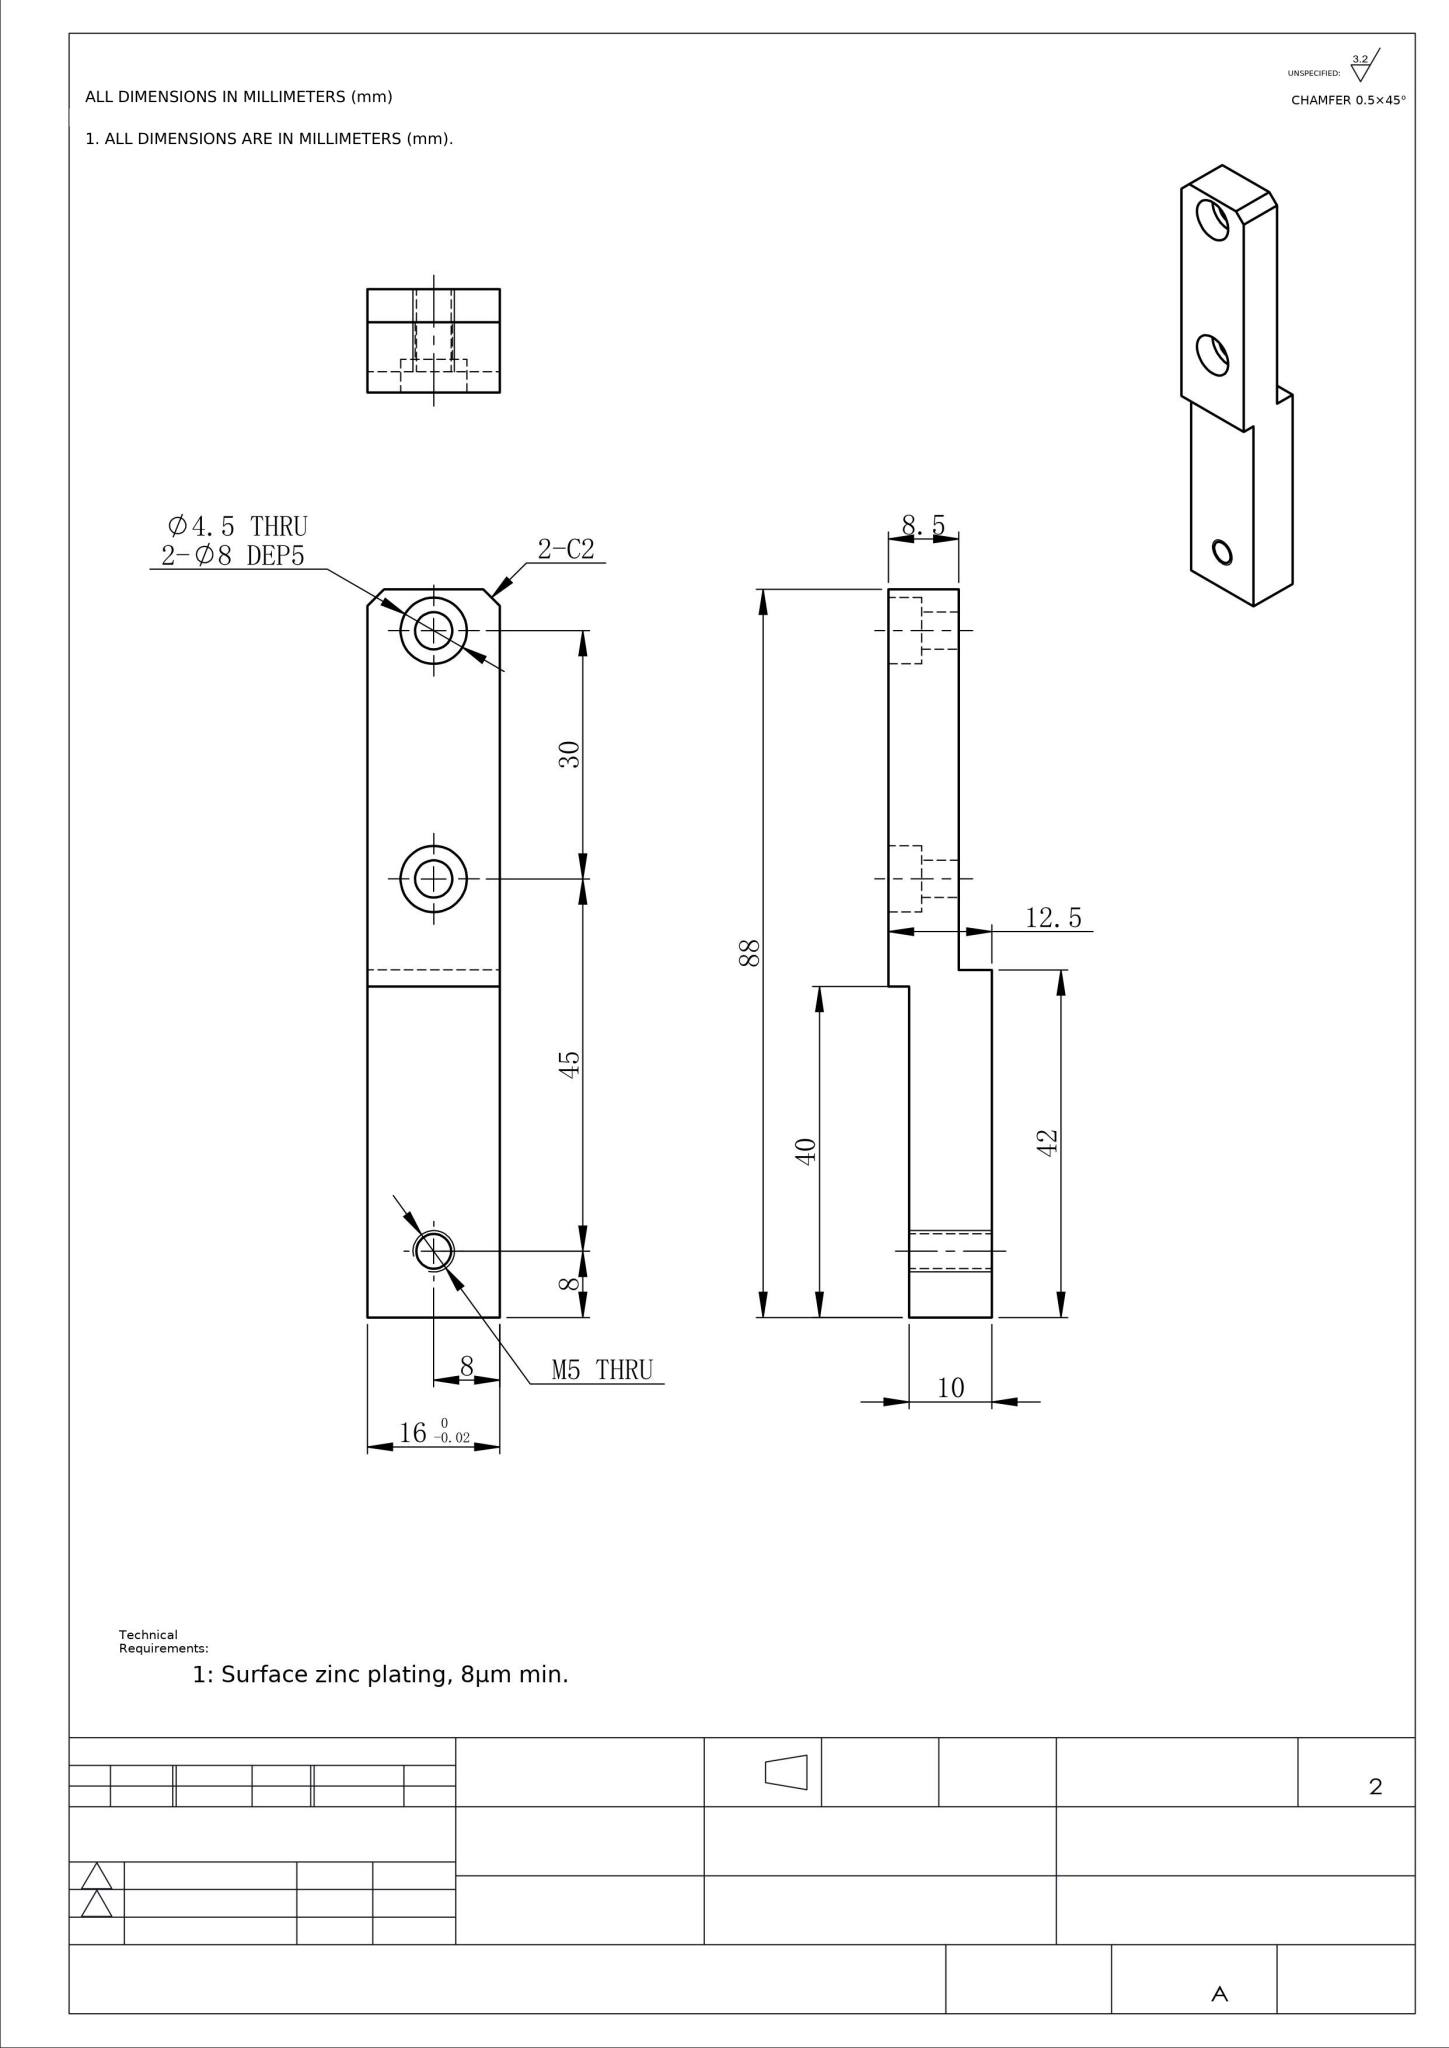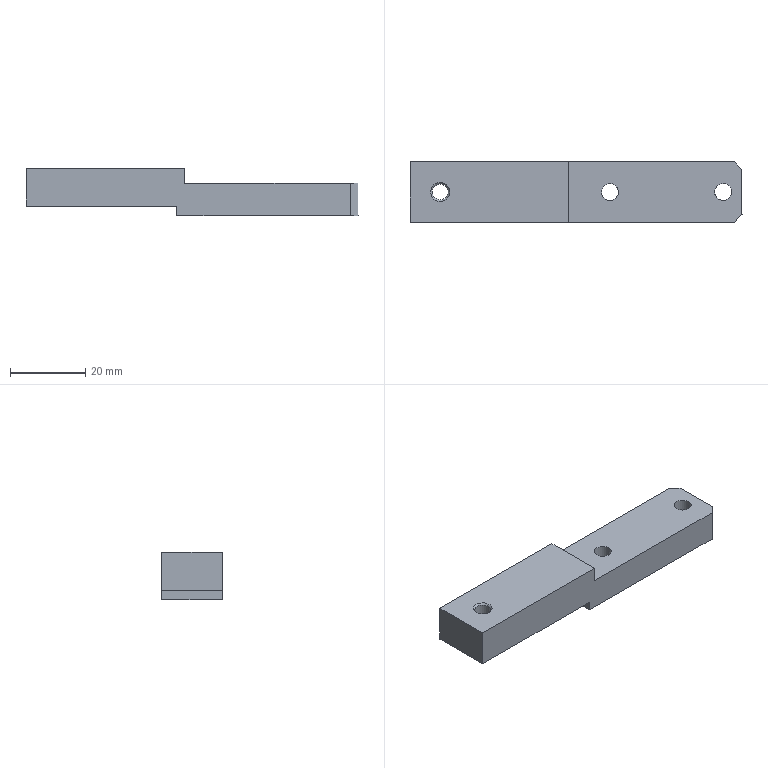Part | NX | mm | Offset Dual-Bore Mounting Bar | 1 solid | 21 faces | box 88 x 16.02 x 12.51 mm | volume 12267 mm3 | plane 14 | cylinder 5 | cone 2 | commonest cylinder face diameters 4.5 x2 8 x2 4.2 x1